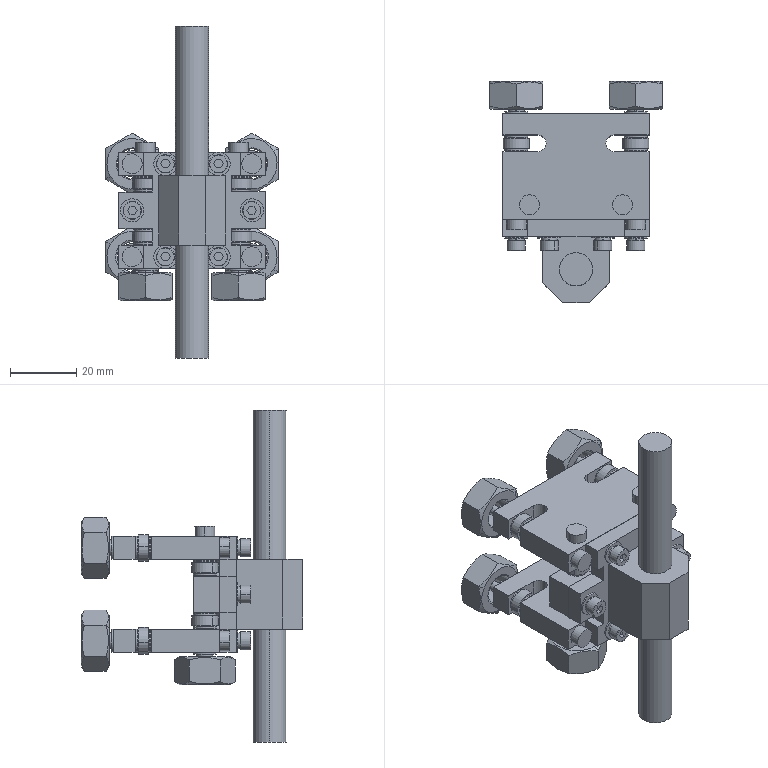Assembly | SolidWorks | mm | 69 component files | 69 solids | 723 faces | box 52 x 66.7 x 100 mm | volume 53480 mm3 | cylinder 324 | plane 307 | cone 68 | torus 24 | commonest cylinder face diameters 3 x92 3.4 x80 7 x56 4.7 x24 5 x16 8 x16 9 x12 6 x12
Bill of materials:
3mmScrewRod | 2 |  | Headed cylindrical pin: a short, wide disc head on one end of a long, plain, straight cylindrical shank with flat ends.
3mmX34ScrewRod | 4 |  | Headed cylindrical pin: a disc head on one end of a long, plain cylindrical shank. It looks much like unnamed part.
618-8BearingHousing | 1 | 6061 Alloy | Block-style bracket: a body with a large vertical through-bore and a chamfered (truncated) bottom profile, joined to a flanged mounting plate with several small through-holes.
BeamSlidingPair | 1 | 6061 Alloy | C-shaped (channel-section) block: two parallel horizontal plates joined by a vertical web along one side. The plates have open-ended U-slots and through-holes, and the web has holes too.
CenterAxis | 1 |  | Plain solid cylindrical rod with flat ends and constant diameter.
GB 93-87-3 | 12 |  | Split ring with a rectangular cross-section and one narrow radial gap, resembling a split washer.
GB_T70.1-2000_SocketHeadCapScrew_M3_12 | 6 |  | Socket-head-cap-screw-like part: a cylindrical head with a hexagonal socket recess, and a plain cylindrical shank with a chamfered tip.
GB_T95-2002FlatWasherC-grade3x0.5 | 28 |  | Thin flat annular washer with a central round hole.
hex nuts, style 1-grades ab gb | 6 |  | Hexagonal nut: a six-sided prism with chamfered corners on both faces and a central round through-bore with a chamfer or countersink at the bore edge.
Roller | 8 |  | Thick cylindrical ring or spacer: a short solid cylinder with a concentric round through-hole.
Mates:
1. distance | Roller-2 face at (-12.097, -8.483, 51.5) dir (0, 0, 1) | BeamSlidingPair-1 face at (23.903, 1.017, 52.5) dir (0, 0, -1)
2. concentric | BeamSlidingPair-1 face at (-12.097, -8.483, 59.5) dir (0, 0, -1) r 1.5 | Roller-2 face at (-12.097, -8.483, 51.5) dir (0, 0, -1) r 1.5
3. concentric | BeamSlidingPair-1 face at (-12.097, -8.483, 59.5) dir (0, 0, -1) r 1.5 | 3mmScrewRod-1 face at (-12.097, -8.483, 59.5) dir (0, 0, -1) r 1.5
4. coincident | BeamSlidingPair-1 face at (23.903, 1.017, 59.5) dir (0, 0, 1) | 3mmScrewRod-1 face at (-12.097, -8.483, 59.5) dir (0, 0, -1)
5. concentric | 3mmX34ScrewRod-1 face at (-16.097, 24.017, 56) dir (0, -1, 0) r 1.5 | Roller-12 face at (-16.097, 8.517, 56) dir (0, 1, 0) r 1.5
6. distance | Roller-12 face at (-16.097, 8.517, 56) dir (0, -1, 0) | BeamSlidingPair-1 face at (-7.097, 7.517, 42) dir (0, 1, 0)
7. parallel | hex nuts, style 1-grades ab gb-4 face at (-24.097, 20.317, 51.381) dir (-1, 0, 0) | BeamSlidingPair-1 face at (-20.097, 1.017, 42) dir (-1, 0, 0)
8. concentric | hex nuts, style 1-grades ab gb-1 face at (-12.097, -8.483, 14.8) dir (0, 0, 1) r 4.5 | 3mmScrewRod-1 face at (-12.097, -8.483, 59.5) dir (0, 0, -1) r 1.5
9. coincident | BeamSlidingPair-1 face at (23.903, -12.983, 42) dir (0, -1, 0) | assembly face at (-12.921, -12.983, 28) dir (0, 1, 0)
10. parallel | hex nuts, style 1-grades ab gb-1 face at (-20.097, -3.864, 14.8) dir (-1, 0, 0) | BeamSlidingPair-1 face at (-20.097, 1.017, 42) dir (-1, 0, 0)
11. concentric | GB_T70.1-2000_SocketHeadCapScrew_M3_12-1 face at (9.903, -22.283, 56) dir (0, -1, 0) r 1.5 | GB_T95-2002FlatWasherC-grade3x0.5-1 face at (9.903, -27.127, 56) dir (0, -1, 0) r 1.7
12. coincident | 618-8BearingHousing-1 face at (-8.097, -17.983, 59.5) dir (0, -1, 0) | GB_T95-2002FlatWasherC-grade3x0.5-1 face at (8.203, -17.983, 56) dir (0, 1, 0)
13. concentric | GB_T70.1-2000_SocketHeadCapScrew_M3_12-1 face at (9.903, -22.283, 56) dir (0, -1, 0) r 1.5 | GB 93-87-3-1 face at (9.903, -18.483, 56) dir (0, -1, 0) r 1.7
14. coincident | GB 93-87-3-1 face at (9.903, -18.483, 56) dir (0, 1, 0) | GB_T95-2002FlatWasherC-grade3x0.5-1 face at (8.203, -18.483, 56) dir (0, -1, 0)
15. coincident | GB_T70.1-2000_SocketHeadCapScrew_M3_12-1 face at (7.522, -19.283, 54.625) dir (0, 1, 0) | GB 93-87-3-1 face at (9.903, -19.283, 56) dir (0, -1, 0)
16. concentric | GB_T70.1-2000_SocketHeadCapScrew_M3_12-2 face at (19.903, -22.283, 42) dir (0, -1, 0) r 1.5 | GB_T95-2002FlatWasherC-grade3x0.5-2 face at (19.903, -27.127, 42) dir (0, -1, 0) r 1.7
17. coincident | 618-8BearingHousing-1 face at (-8.097, -17.983, 59.5) dir (0, -1, 0) | GB_T95-2002FlatWasherC-grade3x0.5-2 face at (19.512, -17.983, 43.654) dir (0, 1, 0)
18. coincident | GB_T95-2002FlatWasherC-grade3x0.5-2 face at (19.512, -18.483, 43.654) dir (0, -1, 0) | GB 93-87-3-2 face at (19.903, -18.483, 42) dir (0, 1, 0)
19. concentric | GB_T70.1-2000_SocketHeadCapScrew_M3_12-2 face at (19.903, -22.283, 42) dir (0, -1, 0) r 1.5 | GB 93-87-3-2 face at (19.903, -18.483, 42) dir (0, -1, 0) r 1.7
20. coincident | GB_T70.1-2000_SocketHeadCapScrew_M3_12-2 face at (19.903, -19.283, 39.25) dir (0, 1, 0) | GB 93-87-3-2 face at (19.903, -19.283, 42) dir (0, -1, 0)
21. concentric | GB_T70.1-2000_SocketHeadCapScrew_M3_12-3 face at (9.903, -22.283, 28) dir (0, -1, 0) r 1.5 | GB_T95-2002FlatWasherC-grade3x0.5-3 face at (9.903, -27.127, 28) dir (0, -1, 0) r 1.7
22. coincident | 618-8BearingHousing-1 face at (-8.097, -17.983, 59.5) dir (0, -1, 0) | GB_T95-2002FlatWasherC-grade3x0.5-3 face at (8.203, -17.983, 28) dir (0, 1, 0)
23. coincident | GB 93-87-3-3 face at (9.903, -18.483, 28) dir (0, 1, 0) | GB_T95-2002FlatWasherC-grade3x0.5-3 face at (8.203, -18.483, 28) dir (0, -1, 0)
24. concentric | GB_T70.1-2000_SocketHeadCapScrew_M3_12-3 face at (9.903, -22.283, 28) dir (0, -1, 0) r 1.5 | GB 93-87-3-3 face at (9.903, -18.483, 28) dir (0, -1, 0) r 1.7
25. coincident | GB_T70.1-2000_SocketHeadCapScrew_M3_12-3 face at (7.522, -19.283, 26.625) dir (0, 1, 0) | GB 93-87-3-3 face at (9.903, -19.283, 28) dir (0, -1, 0)
26. coincident | BeamSlidingPair-1 face at (23.903, -12.983, 42) dir (0, -1, 0) | 618-8BearingHousing-1 face at (22.903, -12.983, 59.5) dir (0, 1, 0)
27. concentric | BeamSlidingPair-1 face at (19.903, -12.983, 42) dir (0, -1, 0) r 1.5 | 618-8BearingHousing-1 face at (19.903, -12.983, 42) dir (0, -1, 0) r 1.5
28. concentric | BeamSlidingPair-1 face at (-16.097, -12.983, 42) dir (0, -1, 0) r 1.5 | 618-8BearingHousing-1 face at (-16.097, -12.983, 42) dir (0, -1, 0) r 1.5
29. concentric | 618-8BearingHousing-1 face at (19.903, -12.983, 42) dir (0, -1, 0) r 1.5 | GB_T70.1-2000_SocketHeadCapScrew_M3_12-2 face at (19.903, -22.283, 42) dir (0, -1, 0) r 1.5
30. concentric | 618-8BearingHousing-1 face at (9.903, -12.983, 56) dir (0, -1, 0) r 1.5 | GB_T70.1-2000_SocketHeadCapScrew_M3_12-1 face at (9.903, -22.283, 56) dir (0, -1, 0) r 1.5
31. concentric | 618-8BearingHousing-1 face at (9.903, -12.983, 28) dir (0, -1, 0) r 1.5 | GB_T70.1-2000_SocketHeadCapScrew_M3_12-3 face at (9.903, -22.283, 28) dir (0, -1, 0) r 1.5
32. concentric | BeamSlidingPair-1 face at (-16.097, -12.983, 56) dir (0, 1, 0) r 1.5 | 3mmX34ScrewRod-1 face at (-16.097, 24.017, 56) dir (0, -1, 0) r 1.5
33. coincident | BeamSlidingPair-1 face at (23.903, -12.983, 42) dir (0, -1, 0) | 3mmX34ScrewRod-1 face at (-16.097, -12.983, 56) dir (0, 1, 0)
34. concentric | 3mmScrewRod-1 face at (-12.097, -8.483, 59.5) dir (0, 0, -1) r 1.5 | GB_T95-2002FlatWasherC-grade3x0.5-10 face at (-12.097, -8.483, 33.145) dir (0, 0, 1) r 1.7
35. coincident | BeamSlidingPair-1 face at (23.903, 1.017, 24.5) dir (0, 0, -1) | GB_T95-2002FlatWasherC-grade3x0.5-10 face at (-13.797, -8.483, 24.5) dir (0, 0, 1)
36. concentric | 3mmScrewRod-1 face at (-12.097, -8.483, 59.5) dir (0, 0, -1) r 1.5 | GB 93-87-3-7 face at (-12.097, -8.483, 23.2) dir (0, 0, 1) r 1.7
37. coincident | GB 93-87-3-7 face at (-12.097, -8.483, 24) dir (0, 0, 1) | GB_T95-2002FlatWasherC-grade3x0.5-10 face at (-13.797, -8.483, 24) dir (0, 0, -1)
38. coincident | hex nuts, style 1-grades ab gb-1 face at (-12.097, 0.7548, 23.2) dir (0, 0, 1) | GB 93-87-3-7 face at (-12.097, -8.483, 23.2) dir (0, 0, -1)
39. concentric | 3mmX34ScrewRod-1 face at (-16.097, 24.017, 56) dir (0, -1, 0) r 1.5 | GB_T95-2002FlatWasherC-grade3x0.5-23 face at (-16.097, 10.373, 56) dir (0, -1, 0) r 1.7
40. coincident | BeamSlidingPair-1 face at (23.903, 19.017, 42) dir (0, 1, 0) | GB_T95-2002FlatWasherC-grade3x0.5-23 face at (-17.346, 19.017, 54.847) dir (0, -1, 0)
41. concentric | 3mmX34ScrewRod-1 face at (-16.097, 24.017, 56) dir (0, -1, 0) r 1.5 | GB 93-87-3-8 face at (-16.097, 19.517, 56) dir (0, 1, 0) r 1.7
42. coincident | GB_T95-2002FlatWasherC-grade3x0.5-23 face at (-17.346, 19.517, 54.847) dir (0, 1, 0) | GB 93-87-3-8 face at (-16.097, 19.517, 56) dir (0, -1, 0)
43. concentric | 3mmX34ScrewRod-1 face at (-16.097, 24.017, 56) dir (0, -1, 0) r 1.5 | hex nuts, style 1-grades ab gb-4 face at (-16.097, 20.317, 56) dir (0, 1, 0) r 4.5
44. coincident | hex nuts, style 1-grades ab gb-4 face at (-24.097, 20.317, 51.381) dir (0, -1, 0) | GB 93-87-3-8 face at (-16.097, 20.317, 56) dir (0, 1, 0)
45. concentric | 3mmX34ScrewRod-1 face at (-16.097, 24.017, 56) dir (0, -1, 0) r 1.5 | GB_T95-2002FlatWasherC-grade3x0.5-27 face at (-16.097, -0.8355, 56) dir (0, -1, 0) r 1.7
46. concentric | 3mmX34ScrewRod-1 face at (-16.097, 24.017, 56) dir (0, -1, 0) r 1.5 | GB_T95-2002FlatWasherC-grade3x0.5-25 face at (-16.097, 3.123, 56) dir (0, -1, 0) r 1.7
47. distance | GB_T95-2002FlatWasherC-grade3x0.5-25 face at (-17.347, 11.767, 54.848) dir (0, -1, 0) | Roller-12 face at (-16.097, 11.517, 56) dir (0, 1, 0)
48. concentric | 3mmScrewRod-1 face at (-12.097, -8.483, 59.5) dir (0, 0, -1) r 1.5 | GB_T95-2002FlatWasherC-grade3x0.5-31 face at (-12.097, -8.483, 60.895) dir (0, 0, 1) r 1.7
49. distance | Roller-2 face at (-12.097, -8.483, 51.5) dir (0, 0, 1) | GB_T95-2002FlatWasherC-grade3x0.5-31 face at (-11.51, -10.078, 51.75) dir (0, 0, -1)
50. concentric | 3mmScrewRod-1 face at (-12.097, -8.483, 59.5) dir (0, 0, -1) r 1.5 | GB_T95-2002FlatWasherC-grade3x0.5-29 face at (-12.097, -8.483, 56.895) dir (0, 0, 1) r 1.7
51. distance | GB_T95-2002FlatWasherC-grade3x0.5-29 face at (-13.341, -9.642, 47.75) dir (0, 0, -1) | BeamSlidingPair-1 face at (-7.097, 1.017, 47.5) dir (0, 0, 1)
52. parallel | GB 93-87-3-8 face at (-16.097, 20.317, 58.351) dir (-0.9659, -0.2588, 0) | assembly plane at (-13.996, -3.75, 0) dir (0.9659, 0.2588, 0)
53. concentric | 618-8BearingHousing-1 face at (1.903, -27.983, 59.5) dir (0, 0, -1) r 5 | CenterAxis-1 face at (1.903, -27.983, 97.5) dir (0, 0, -1) r 5
54. distance | CenterAxis-1 face at (1.903, -27.983, 97.5) dir (0, 0, 1) | 618-8BearingHousing-1 face at (1.903, -15.483, 52.5) dir (0, 0, 1)